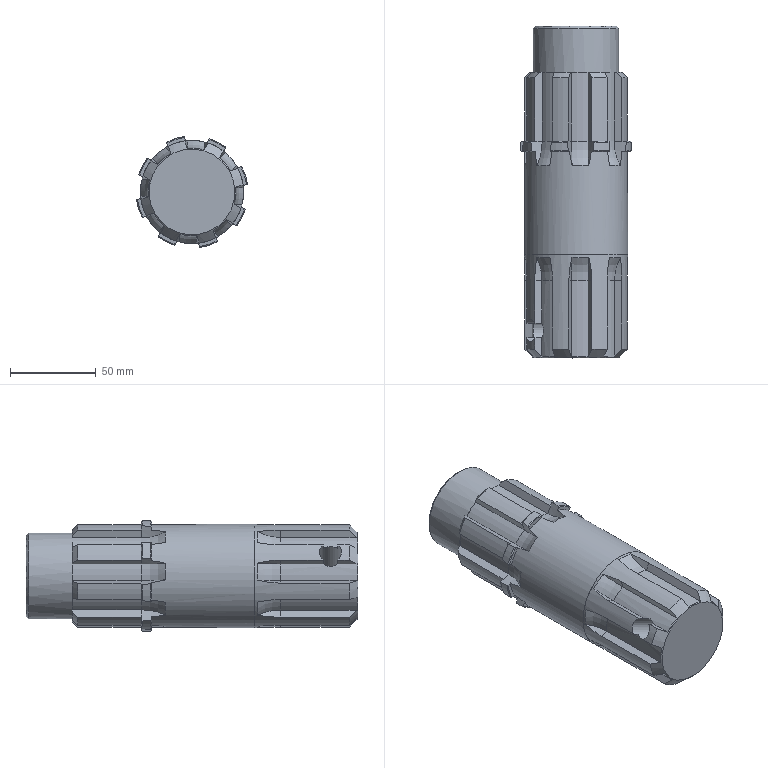Component | NX | LOWER_SHAFT | 1 solid | 168 faces | volume 469715 mm3 | cone 58 | plane 56 | cylinder 38 | torus 16 | commonest cylinder face diameters 60 x9 51 x8 65 x8 50.5 x8 59.98 x3 50 x1 13 x1